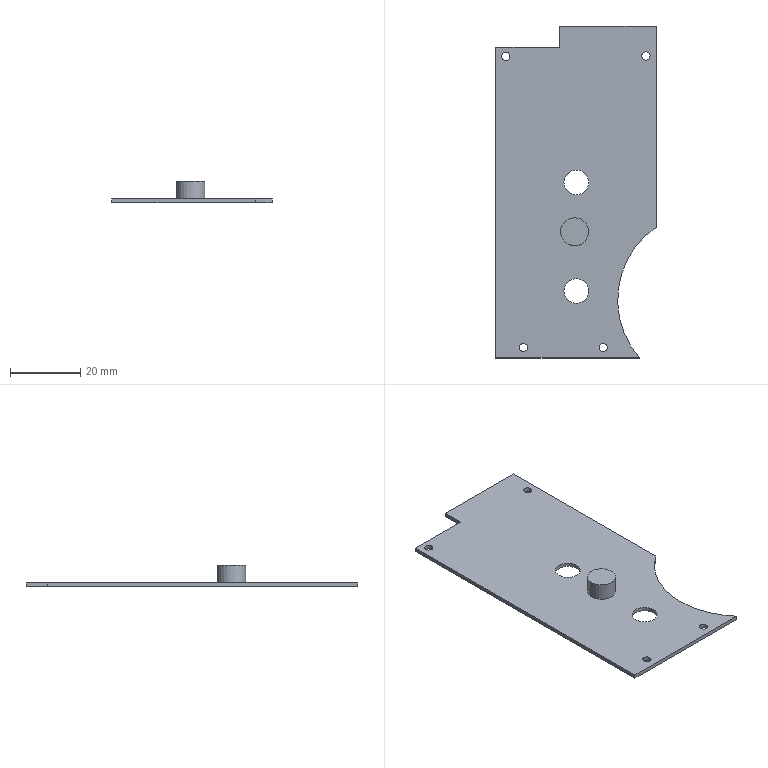Component | NX | PCB_LARGE | 1 solid | 17 faces | volume 4603 mm3 | plane 9 | cylinder 8 | commonest cylinder face diameters 2.35 x4 7.09 x2 50.233 x1 8 x1